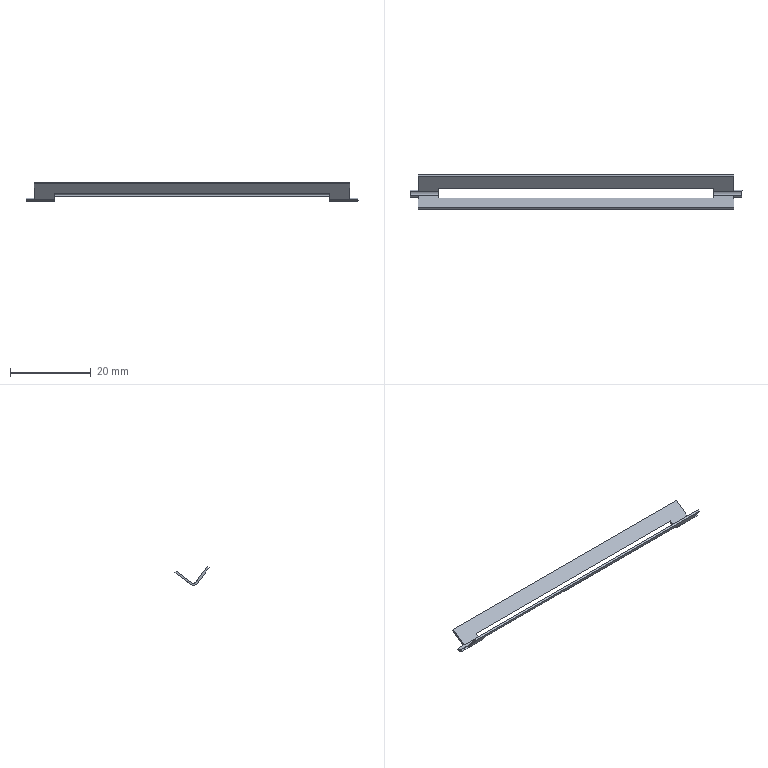Component | SolidWorks | ToolHolderAssembly-1_Blade-1 | 1 solid | 28 faces | box 82 x 8.4 x 4.59 mm | volume 284 mm3 | plane 24 | cylinder 4 | commonest cylinder face diameters 1.5 x2 2.5 x2
STEP:
#1=COLOUR_RGB('',0.7922,0.8196,0.9333);
#2=FILL_AREA_STYLE_COLOUR('',#1);
#3=FILL_AREA_STYLE('',(#2));
#4=SURFACE_STYLE_FILL_AREA(#3);
#5=SURFACE_SIDE_STYLE('',(#4));
#6=SURFACE_STYLE_USAGE(.BOTH.,#5);
#7=PRESENTATION_STYLE_ASSIGNMENT((#6));
#8=CARTESIAN_POINT('',(-4.579,0.3269,5.509));
#9=VERTEX_POINT('',#8);
#10=CARTESIAN_POINT('',(-7.257,0.3269,5.509));
#11=VERTEX_POINT('',#10);
#12=CARTESIAN_POINT('',(-7.257,0.3269,5.509));
#13=DIRECTION('',(-1.,0.,-0.));
#14=VECTOR('',#13,39.37);
#15=LINE('',#12,#14);
#16=EDGE_CURVE('',#9,#11,#15,.T.);
#17=ORIENTED_EDGE('',*,*,#16,.T.);
#18=CARTESIAN_POINT('',(-7.257,0.268,5.465));
#19=VERTEX_POINT('',#18);
#20=CARTESIAN_POINT('',(-7.257,0.2954,5.486));
#21=DIRECTION('',(0.,-0.799,-0.6013));
#22=VECTOR('',#21,39.37);
#23=LINE('',#20,#22);
#24=EDGE_CURVE('',#11,#19,#23,.T.);
#25=ORIENTED_EDGE('',*,*,#24,.T.);
#26=CARTESIAN_POINT('',(-7.453,0.268,5.465));
#27=VERTEX_POINT('',#26);
#28=CARTESIAN_POINT('',(-4.304,0.268,5.465));
#29=DIRECTION('',(-1.,0.,-0.));
#30=VECTOR('',#29,39.37);
#31=LINE('',#28,#30);
#32=EDGE_CURVE('',#19,#27,#31,.T.);
#33=ORIENTED_EDGE('',*,*,#32,.T.);
#34=CARTESIAN_POINT('',(-7.453,0.4174,5.577));
#35=VERTEX_POINT('',#34);
#36=CARTESIAN_POINT('',(-7.453,0.4174,5.577));
#37=DIRECTION('',(0.,-0.799,-0.6013));
#38=VECTOR('',#37,39.37);
#39=LINE('',#36,#38);
#40=EDGE_CURVE('',#35,#27,#39,.T.);
#41=ORIENTED_EDGE('',*,*,#40,.F.);
#42=CARTESIAN_POINT('',(-4.383,0.4174,5.577));
#43=VERTEX_POINT('',#42);
#44=CARTESIAN_POINT('',(-4.304,0.4174,5.577));
#45=DIRECTION('',(-1.,0.,-0.));
#46=VECTOR('',#45,39.37);
#47=LINE('',#44,#46);
#48=EDGE_CURVE('',#43,#35,#47,.T.);
#49=ORIENTED_EDGE('',*,*,#48,.F.);
#50=CARTESIAN_POINT('',(-4.383,0.268,5.465));
#51=VERTEX_POINT('',#50);
#52=CARTESIAN_POINT('',(-4.383,0.268,5.465));
#53=DIRECTION('',(-0.,0.799,0.6013));
#54=VECTOR('',#53,39.37);
#55=LINE('',#52,#54);
#56=EDGE_CURVE('',#51,#43,#55,.T.);
#57=ORIENTED_EDGE('',*,*,#56,.F.);
#58=CARTESIAN_POINT('',(-4.579,0.268,5.465));
#59=VERTEX_POINT('',#58);
#60=CARTESIAN_POINT('',(-4.304,0.268,5.465));
#61=DIRECTION('',(-1.,0.,-0.));
#62=VECTOR('',#61,39.37);
#63=LINE('',#60,#62);
#64=EDGE_CURVE('',#51,#59,#63,.T.);
#65=ORIENTED_EDGE('',*,*,#64,.T.);
#66=CARTESIAN_POINT('',(-4.579,0.1912,5.407));
#67=DIRECTION('',(-0.,0.799,0.6013));
#68=VECTOR('',#67,39.37);
#69=LINE('',#66,#68);
#70=EDGE_CURVE('',#59,#9,#69,.T.);
#71=ORIENTED_EDGE('',*,*,#70,.T.);
#72=EDGE_LOOP('',(#17,#25,#33,#41,#49,#57,#65,#71));
#73=FACE_OUTER_BOUND('',#72,.T.);
#74=CARTESIAN_POINT('',(-4.304,0.268,5.465));
#75=DIRECTION('',(-0.,-0.6013,0.799));
#76=DIRECTION('',(1.,-0.,0.));
#77=AXIS2_PLACEMENT_3D('',#74,#75,#76);
#78=PLANE('',#77);
#79=ADVANCED_FACE('',(#73),#78,.F.);
#80=CARTESIAN_POINT('',(-7.257,0.2878,5.505));
#81=VERTEX_POINT('',#80);
#82=CARTESIAN_POINT('',(-7.257,0.2562,5.481));
#83=VERTEX_POINT('',#82);
#84=CARTESIAN_POINT('',(-7.257,0.2315,5.462));
#85=DIRECTION('',(0.,-0.799,-0.6013));
#86=VECTOR('',#85,39.37);
#87=LINE('',#84,#86);
#88=EDGE_CURVE('',#81,#83,#87,.T.);
#89=ORIENTED_EDGE('',*,*,#88,.F.);
#90=CARTESIAN_POINT('',(-4.579,0.2878,5.505));
#91=VERTEX_POINT('',#90);
#92=CARTESIAN_POINT('',(-4.304,0.2878,5.505));
#93=DIRECTION('',(1.,-0.,0.));
#94=VECTOR('',#93,39.37);
#95=LINE('',#92,#94);
#96=EDGE_CURVE('',#81,#91,#95,.T.);
#97=ORIENTED_EDGE('',*,*,#96,.T.);
#98=CARTESIAN_POINT('',(-4.579,0.2562,5.481));
#99=VERTEX_POINT('',#98);
#100=CARTESIAN_POINT('',(-4.579,0.2315,5.462));
#101=DIRECTION('',(-0.,0.799,0.6013));
#102=VECTOR('',#101,39.37);
#103=LINE('',#100,#102);
#104=EDGE_CURVE('',#99,#91,#103,.T.);
#105=ORIENTED_EDGE('',*,*,#104,.F.);
#106=CARTESIAN_POINT('',(-4.383,0.2562,5.481));
#107=VERTEX_POINT('',#106);
#108=CARTESIAN_POINT('',(-4.304,0.2562,5.481));
#109=DIRECTION('',(-1.,0.,-0.));
#110=VECTOR('',#109,39.37);
#111=LINE('',#108,#110);
#112=EDGE_CURVE('',#107,#99,#111,.T.);
#113=ORIENTED_EDGE('',*,*,#112,.F.);
#114=CARTESIAN_POINT('',(-4.383,0.4056,5.593));
#115=VERTEX_POINT('',#114);
#116=CARTESIAN_POINT('',(-4.383,0.4056,5.593));
#117=DIRECTION('',(0.,-0.799,-0.6013));
#118=VECTOR('',#117,39.37);
#119=LINE('',#116,#118);
#120=EDGE_CURVE('',#115,#107,#119,.T.);
#121=ORIENTED_EDGE('',*,*,#120,.F.);
#122=CARTESIAN_POINT('',(-7.453,0.4056,5.593));
#123=VERTEX_POINT('',#122);
#124=CARTESIAN_POINT('',(-4.304,0.4056,5.593));
#125=DIRECTION('',(-1.,0.,-0.));
#126=VECTOR('',#125,39.37);
#127=LINE('',#124,#126);
#128=EDGE_CURVE('',#115,#123,#127,.T.);
#129=ORIENTED_EDGE('',*,*,#128,.T.);
#130=CARTESIAN_POINT('',(-7.453,0.2562,5.481));
#131=VERTEX_POINT('',#130);
#132=CARTESIAN_POINT('',(-7.453,0.2562,5.481));
#133=DIRECTION('',(-0.,0.799,0.6013));
#134=VECTOR('',#133,39.37);
#135=LINE('',#132,#134);
#136=EDGE_CURVE('',#131,#123,#135,.T.);
#137=ORIENTED_EDGE('',*,*,#136,.F.);
#138=CARTESIAN_POINT('',(-4.304,0.2562,5.481));
#139=DIRECTION('',(-1.,0.,-0.));
#140=VECTOR('',#139,39.37);
#141=LINE('',#138,#140);
#142=EDGE_CURVE('',#83,#131,#141,.T.);
#143=ORIENTED_EDGE('',*,*,#142,.F.);
#144=EDGE_LOOP('',(#89,#97,#105,#113,#121,#129,#137,#143));
#145=FACE_OUTER_BOUND('',#144,.T.);
#146=CARTESIAN_POINT('',(-4.304,0.2562,5.481));
#147=DIRECTION('',(-0.,-0.6013,0.799));
#148=DIRECTION('',(1.,-0.,0.));
#149=AXIS2_PLACEMENT_3D('',#146,#147,#148);
#150=PLANE('',#149);
#151=ADVANCED_FACE('',(#145),#150,.T.);
#152=CARTESIAN_POINT('',(-4.579,0.191,5.518));
#153=VERTEX_POINT('',#152);
#154=CARTESIAN_POINT('',(-4.579,0.2148,5.487));
#155=VERTEX_POINT('',#154);
#156=CARTESIAN_POINT('',(-4.579,0.2334,5.462));
#157=DIRECTION('',(0.,0.6013,-0.799));
#158=VECTOR('',#157,39.37);
#159=LINE('',#156,#158);
#160=EDGE_CURVE('',#153,#155,#159,.T.);
#161=ORIENTED_EDGE('',*,*,#160,.F.);
#162=CARTESIAN_POINT('',(-7.257,0.191,5.518));
#163=VERTEX_POINT('',#162);
#164=CARTESIAN_POINT('',(-4.304,0.191,5.518));
#165=DIRECTION('',(-1.,0.,-0.));
#166=VECTOR('',#165,39.37);
#167=LINE('',#164,#166);
#168=EDGE_CURVE('',#153,#163,#167,.T.);
#169=ORIENTED_EDGE('',*,*,#168,.T.);
#170=CARTESIAN_POINT('',(-7.257,0.2148,5.487));
#171=VERTEX_POINT('',#170);
#172=CARTESIAN_POINT('',(-7.257,0.2334,5.462));
#173=DIRECTION('',(-0.,-0.6013,0.799));
#174=VECTOR('',#173,39.37);
#175=LINE('',#172,#174);
#176=EDGE_CURVE('',#171,#163,#175,.T.);
#177=ORIENTED_EDGE('',*,*,#176,.F.);
#178=CARTESIAN_POINT('',(-7.453,0.2148,5.487));
#179=VERTEX_POINT('',#178);
#180=CARTESIAN_POINT('',(-4.304,0.2148,5.487));
#181=DIRECTION('',(-1.,0.,-0.));
#182=VECTOR('',#181,39.37);
#183=LINE('',#180,#182);
#184=EDGE_CURVE('',#171,#179,#183,.T.);
#185=ORIENTED_EDGE('',*,*,#184,.T.);
#186=CARTESIAN_POINT('',(-7.453,0.1024,5.636));
#187=VERTEX_POINT('',#186);
#188=CARTESIAN_POINT('',(-7.453,0.1024,5.636));
#189=DIRECTION('',(0.,0.6013,-0.799));
#190=VECTOR('',#189,39.37);
#191=LINE('',#188,#190);
#192=EDGE_CURVE('',#187,#179,#191,.T.);
#193=ORIENTED_EDGE('',*,*,#192,.F.);
#194=CARTESIAN_POINT('',(-4.383,0.1024,5.636));
#195=VERTEX_POINT('',#194);
#196=CARTESIAN_POINT('',(-4.304,0.1024,5.636));
#197=DIRECTION('',(-1.,0.,-0.));
#198=VECTOR('',#197,39.37);
#199=LINE('',#196,#198);
#200=EDGE_CURVE('',#195,#187,#199,.T.);
#201=ORIENTED_EDGE('',*,*,#200,.F.);
#202=CARTESIAN_POINT('',(-4.383,0.2148,5.487));
#203=VERTEX_POINT('',#202);
#204=CARTESIAN_POINT('',(-4.383,0.2148,5.487));
#205=DIRECTION('',(-0.,-0.6013,0.799));
#206=VECTOR('',#205,39.37);
#207=LINE('',#204,#206);
#208=EDGE_CURVE('',#203,#195,#207,.T.);
#209=ORIENTED_EDGE('',*,*,#208,.F.);
#210=CARTESIAN_POINT('',(-4.304,0.2148,5.487));
#211=DIRECTION('',(-1.,0.,-0.));
#212=VECTOR('',#211,39.37);
#213=LINE('',#210,#212);
#214=EDGE_CURVE('',#203,#155,#213,.T.);
#215=ORIENTED_EDGE('',*,*,#214,.T.);
#216=EDGE_LOOP('',(#161,#169,#177,#185,#193,#201,#209,#215));
#217=FACE_OUTER_BOUND('',#216,.T.);
#218=CARTESIAN_POINT('',(-4.304,0.1024,5.636));
#219=DIRECTION('',(-0.,0.799,0.6013));
#220=DIRECTION('',(-1.,0.,-0.));
#221=AXIS2_PLACEMENT_3D('',#218,#219,#220);
#222=PLANE('',#221);
#223=ADVANCED_FACE('',(#217),#222,.T.);
#224=CARTESIAN_POINT('',(-7.257,0.1548,5.534));
#225=VERTEX_POINT('',#224);
#226=CARTESIAN_POINT('',(-4.579,0.1548,5.534));
#227=VERTEX_POINT('',#226);
#228=CARTESIAN_POINT('',(-4.579,0.1548,5.534));
#229=DIRECTION('',(1.,-0.,0.));
#230=VECTOR('',#229,39.37);
#231=LINE('',#228,#230);
#232=EDGE_CURVE('',#225,#227,#231,.T.);
#233=ORIENTED_EDGE('',*,*,#232,.T.);
#234=CARTESIAN_POINT('',(-4.579,0.1991,5.475));
#235=VERTEX_POINT('',#234);
#236=CARTESIAN_POINT('',(-4.579,0.1785,5.502));
#237=DIRECTION('',(0.,0.6013,-0.799));
#238=VECTOR('',#237,39.37);
#239=LINE('',#236,#238);
#240=EDGE_CURVE('',#227,#235,#239,.T.);
#241=ORIENTED_EDGE('',*,*,#240,.T.);
#242=CARTESIAN_POINT('',(-4.383,0.1991,5.475));
#243=VERTEX_POINT('',#242);
#244=CARTESIAN_POINT('',(-4.304,0.1991,5.475));
#245=DIRECTION('',(-1.,0.,-0.));
#246=VECTOR('',#245,39.37);
#247=LINE('',#244,#246);
#248=EDGE_CURVE('',#243,#235,#247,.T.);
#249=ORIENTED_EDGE('',*,*,#248,.F.);
#250=CARTESIAN_POINT('',(-4.383,0.08665,5.624));
#251=VERTEX_POINT('',#250);
#252=CARTESIAN_POINT('',(-4.383,0.08665,5.624));
#253=DIRECTION('',(0.,0.6013,-0.799));
#254=VECTOR('',#253,39.37);
#255=LINE('',#252,#254);
#256=EDGE_CURVE('',#251,#243,#255,.T.);
#257=ORIENTED_EDGE('',*,*,#256,.F.);
#258=CARTESIAN_POINT('',(-7.453,0.08665,5.624));
#259=VERTEX_POINT('',#258);
#260=CARTESIAN_POINT('',(-4.304,0.08665,5.624));
#261=DIRECTION('',(-1.,0.,-0.));
#262=VECTOR('',#261,39.37);
#263=LINE('',#260,#262);
#264=EDGE_CURVE('',#251,#259,#263,.T.);
#265=ORIENTED_EDGE('',*,*,#264,.T.);
#266=CARTESIAN_POINT('',(-7.453,0.1991,5.475));
#267=VERTEX_POINT('',#266);
#268=CARTESIAN_POINT('',(-7.453,0.1991,5.475));
#269=DIRECTION('',(-0.,-0.6013,0.799));
#270=VECTOR('',#269,39.37);
#271=LINE('',#268,#270);
#272=EDGE_CURVE('',#267,#259,#271,.T.);
#273=ORIENTED_EDGE('',*,*,#272,.F.);
#274=CARTESIAN_POINT('',(-7.257,0.1991,5.475));
#275=VERTEX_POINT('',#274);
#276=CARTESIAN_POINT('',(-4.304,0.1991,5.475));
#277=DIRECTION('',(-1.,0.,-0.));
#278=VECTOR('',#277,39.37);
#279=LINE('',#276,#278);
#280=EDGE_CURVE('',#275,#267,#279,.T.);
#281=ORIENTED_EDGE('',*,*,#280,.F.);
#282=CARTESIAN_POINT('',(-7.257,0.2569,5.398));
#283=DIRECTION('',(-0.,-0.6013,0.799));
#284=VECTOR('',#283,39.37);
#285=LINE('',#282,#284);
#286=EDGE_CURVE('',#275,#225,#285,.T.);
#287=ORIENTED_EDGE('',*,*,#286,.T.);
#288=EDGE_LOOP('',(#233,#241,#249,#257,#265,#273,#281,#287));
#289=FACE_OUTER_BOUND('',#288,.T.);
#290=CARTESIAN_POINT('',(-4.304,0.08665,5.624));
#291=DIRECTION('',(-0.,0.799,0.6013));
#292=DIRECTION('',(-1.,0.,-0.));
#293=AXIS2_PLACEMENT_3D('',#290,#291,#292);
#294=PLANE('',#293);
#295=ADVANCED_FACE('',(#289),#294,.F.);
#296=ORIENTED_EDGE('',*,*,#184,.F.);
#297=CARTESIAN_POINT('',(-7.257,0.2384,5.504));
#298=DIRECTION('',(1.,-0.,0.));
#299=DIRECTION('',(0.,-0.799,-0.6013));
#300=AXIS2_PLACEMENT_3D('',#297,#298,#299);
#301=CIRCLE('',#300,0.02953);
#302=EDGE_CURVE('',#171,#83,#301,.T.);
#303=ORIENTED_EDGE('',*,*,#302,.T.);
#304=ORIENTED_EDGE('',*,*,#142,.T.);
#305=CARTESIAN_POINT('',(-7.532,0.2562,5.481));
#306=VERTEX_POINT('',#305);
#307=CARTESIAN_POINT('',(-7.453,0.2562,5.481));
#308=DIRECTION('',(-1.,0.,-0.));
#309=VECTOR('',#308,39.37);
#310=LINE('',#307,#309);
#311=EDGE_CURVE('',#131,#306,#310,.T.);
#312=ORIENTED_EDGE('',*,*,#311,.T.);
#313=CARTESIAN_POINT('',(-7.532,0.2148,5.487));
#314=VERTEX_POINT('',#313);
#315=CARTESIAN_POINT('',(-7.532,0.2384,5.504));
#316=DIRECTION('',(1.,-0.,0.));
#317=DIRECTION('',(0.,0.799,0.6013));
#318=AXIS2_PLACEMENT_3D('',#315,#316,#317);
#319=CIRCLE('',#318,0.02953);
#320=EDGE_CURVE('',#314,#306,#319,.T.);
#321=ORIENTED_EDGE('',*,*,#320,.F.);
#322=CARTESIAN_POINT('',(-7.453,0.2148,5.487));
#323=DIRECTION('',(-1.,0.,-0.));
#324=VECTOR('',#323,39.37);
#325=LINE('',#322,#324);
#326=EDGE_CURVE('',#179,#314,#325,.T.);
#327=ORIENTED_EDGE('',*,*,#326,.F.);
#328=EDGE_LOOP('',(#296,#303,#304,#312,#321,#327));
#329=FACE_OUTER_BOUND('',#328,.T.);
#330=CARTESIAN_POINT('',(-4.304,0.2384,5.504));
#331=DIRECTION('',(-1.,0.,-0.));
#332=DIRECTION('',(0.,-0.799,-0.6013));
#333=AXIS2_PLACEMENT_3D('',#330,#331,#332);
#334=CYLINDRICAL_SURFACE('',#333,0.02953);
#335=ADVANCED_FACE('',(#329),#334,.F.);
#336=ORIENTED_EDGE('',*,*,#112,.T.);
#337=CARTESIAN_POINT('',(-4.579,0.2384,5.504));
#338=DIRECTION('',(-1.,0.,-0.));
#339=DIRECTION('',(0.,0.799,0.6013));
#340=AXIS2_PLACEMENT_3D('',#337,#338,#339);
#341=CIRCLE('',#340,0.02953);
#342=EDGE_CURVE('',#99,#155,#341,.T.);
#343=ORIENTED_EDGE('',*,*,#342,.T.);
#344=ORIENTED_EDGE('',*,*,#214,.F.);
#345=CARTESIAN_POINT('',(-4.304,0.2148,5.487));
#346=VERTEX_POINT('',#345);
#347=CARTESIAN_POINT('',(-4.304,0.2148,5.487));
#348=DIRECTION('',(-1.,0.,-0.));
#349=VECTOR('',#348,39.37);
#350=LINE('',#347,#349);
#351=EDGE_CURVE('',#346,#203,#350,.T.);
#352=ORIENTED_EDGE('',*,*,#351,.F.);
#353=CARTESIAN_POINT('',(-4.304,0.2562,5.481));
#354=VERTEX_POINT('',#353);
#355=CARTESIAN_POINT('',(-4.304,0.2384,5.504));
#356=DIRECTION('',(1.,-0.,0.));
#357=DIRECTION('',(0.,0.799,0.6013));
#358=AXIS2_PLACEMENT_3D('',#355,#356,#357);
#359=CIRCLE('',#358,0.02953);
#360=EDGE_CURVE('',#346,#354,#359,.T.);
#361=ORIENTED_EDGE('',*,*,#360,.T.);
#362=CARTESIAN_POINT('',(-4.304,0.2562,5.481));
#363=DIRECTION('',(-1.,0.,-0.));
#364=VECTOR('',#363,39.37);
#365=LINE('',#362,#364);
#366=EDGE_CURVE('',#354,#107,#365,.T.);
#367=ORIENTED_EDGE('',*,*,#366,.T.);
#368=EDGE_LOOP('',(#336,#343,#344,#352,#361,#367));
#369=FACE_OUTER_BOUND('',#368,.T.);
#370=CARTESIAN_POINT('',(-4.304,0.2384,5.504));
#371=DIRECTION('',(-1.,0.,-0.));
#372=DIRECTION('',(0.,-0.799,-0.6013));
#373=AXIS2_PLACEMENT_3D('',#370,#371,#372);
#374=CYLINDRICAL_SURFACE('',#373,0.02953);
#375=ADVANCED_FACE('',(#369),#374,.F.);
#376=CARTESIAN_POINT('',(-7.257,0.2384,5.504));
#377=DIRECTION('',(1.,-0.,0.));
#378=DIRECTION('',(0.,-0.799,-0.6013));
#379=AXIS2_PLACEMENT_3D('',#376,#377,#378);
#380=CIRCLE('',#379,0.04921);
#381=EDGE_CURVE('',#275,#19,#380,.T.);
#382=ORIENTED_EDGE('',*,*,#381,.F.);
#383=ORIENTED_EDGE('',*,*,#280,.T.);
#384=CARTESIAN_POINT('',(-7.532,0.1991,5.475));
#385=VERTEX_POINT('',#384);
#386=CARTESIAN_POINT('',(-7.453,0.1991,5.475));
#387=DIRECTION('',(-1.,0.,-0.));
#388=VECTOR('',#387,39.37);
#389=LINE('',#386,#388);
#390=EDGE_CURVE('',#267,#385,#389,.T.);
#391=ORIENTED_EDGE('',*,*,#390,.T.);
#392=CARTESIAN_POINT('',(-7.532,0.268,5.465));
#393=VERTEX_POINT('',#392);
#394=CARTESIAN_POINT('',(-7.532,0.2384,5.504));
#395=DIRECTION('',(1.,-0.,0.));
#396=DIRECTION('',(0.,-0.799,-0.6013));
#397=AXIS2_PLACEMENT_3D('',#394,#395,#396);
#398=CIRCLE('',#397,0.04921);
#399=EDGE_CURVE('',#385,#393,#398,.T.);
#400=ORIENTED_EDGE('',*,*,#399,.T.);
#401=CARTESIAN_POINT('',(-7.453,0.268,5.465));
#402=DIRECTION('',(-1.,0.,-0.));
#403=VECTOR('',#402,39.37);
#404=LINE('',#401,#403);
#405=EDGE_CURVE('',#27,#393,#404,.T.);
#406=ORIENTED_EDGE('',*,*,#405,.F.);
#407=ORIENTED_EDGE('',*,*,#32,.F.);
#408=EDGE_LOOP('',(#382,#383,#391,#400,#406,#407));
#409=FACE_OUTER_BOUND('',#408,.T.);
#410=CARTESIAN_POINT('',(-4.304,0.2384,5.504));
#411=DIRECTION('',(-1.,0.,-0.));
#412=DIRECTION('',(0.,-0.799,-0.6013));
#413=AXIS2_PLACEMENT_3D('',#410,#411,#412);
#414=CYLINDRICAL_SURFACE('',#413,0.04921);
#415=ADVANCED_FACE('',(#409),#414,.T.);
#416=CARTESIAN_POINT('',(-4.579,0.2384,5.504));
#417=DIRECTION('',(-1.,0.,-0.));
#418=DIRECTION('',(0.,-0.799,-0.6013));
#419=AXIS2_PLACEMENT_3D('',#416,#417,#418);
#420=CIRCLE('',#419,0.04921);
#421=EDGE_CURVE('',#59,#235,#420,.T.);
#422=ORIENTED_EDGE('',*,*,#421,.F.);
#423=ORIENTED_EDGE('',*,*,#64,.F.);
#424=CARTESIAN_POINT('',(-4.304,0.268,5.465));
#425=VERTEX_POINT('',#424);
#426=CARTESIAN_POINT('',(-4.304,0.268,5.465));
#427=DIRECTION('',(-1.,0.,-0.));
#428=VECTOR('',#427,39.37);
#429=LINE('',#426,#428);
#430=EDGE_CURVE('',#425,#51,#429,.T.);
#431=ORIENTED_EDGE('',*,*,#430,.F.);
#432=CARTESIAN_POINT('',(-4.304,0.1991,5.475));
#433=VERTEX_POINT('',#432);
#434=CARTESIAN_POINT('',(-4.304,0.2384,5.504));
#435=DIRECTION('',(1.,-0.,0.));
#436=DIRECTION('',(0.,-0.799,-0.6013));
#437=AXIS2_PLACEMENT_3D('',#434,#435,#436);
#438=CIRCLE('',#437,0.04921);
#439=EDGE_CURVE('',#433,#425,#438,.T.);
#440=ORIENTED_EDGE('',*,*,#439,.F.);
#441=CARTESIAN_POINT('',(-4.304,0.1991,5.475));
#442=DIRECTION('',(-1.,0.,-0.));
#443=VECTOR('',#442,39.37);
#444=LINE('',#441,#443);
#445=EDGE_CURVE('',#433,#243,#444,.T.);
#446=ORIENTED_EDGE('',*,*,#445,.T.);
#447=ORIENTED_EDGE('',*,*,#248,.T.);
#448=EDGE_LOOP('',(#422,#423,#431,#440,#446,#447));
#449=FACE_OUTER_BOUND('',#448,.T.);
#450=CARTESIAN_POINT('',(-4.304,0.2384,5.504));
#451=DIRECTION('',(-1.,0.,-0.));
#452=DIRECTION('',(0.,-0.799,-0.6013));
#453=AXIS2_PLACEMENT_3D('',#450,#451,#452);
#454=CYLINDRICAL_SURFACE('',#453,0.04921);
#455=ADVANCED_FACE('',(#449),#454,.T.);
#456=ORIENTED_EDGE('',*,*,#48,.T.);
#457=CARTESIAN_POINT('',(-7.453,0.4056,5.593));
#458=DIRECTION('',(0.,0.6013,-0.799));
#459=VECTOR('',#458,39.37);
#460=LINE('',#457,#459);
#461=EDGE_CURVE('',#123,#35,#460,.T.);
#462=ORIENTED_EDGE('',*,*,#461,.F.);
#463=ORIENTED_EDGE('',*,*,#128,.F.);
#464=CARTESIAN_POINT('',(-4.383,0.4174,5.577));
#465=DIRECTION('',(-0.,-0.6013,0.799));
#466=VECTOR('',#465,39.37);
#467=LINE('',#464,#466);
#468=EDGE_CURVE('',#43,#115,#467,.T.);
#469=ORIENTED_EDGE('',*,*,#468,.F.);
#470=EDGE_LOOP('',(#456,#462,#463,#469));
#471=FACE_OUTER_BOUND('',#470,.T.);
#472=CARTESIAN_POINT('',(-4.304,0.4056,5.593));
#473=DIRECTION('',(-0.,0.799,0.6013));
#474=DIRECTION('',(-1.,0.,-0.));
#475=AXIS2_PLACEMENT_3D('',#472,#473,#474);
#476=PLANE('',#475);
#477=ADVANCED_FACE('',(#471),#476,.T.);
#478=ORIENTED_EDGE('',*,*,#200,.T.);
#479=CARTESIAN_POINT('',(-7.453,0.08665,5.624));
#480=DIRECTION('',(-0.,0.799,0.6013));
#481=VECTOR('',#480,39.37);
#482=LINE('',#479,#481);
#483=EDGE_CURVE('',#259,#187,#482,.T.);
#484=ORIENTED_EDGE('',*,*,#483,.F.);
#485=ORIENTED_EDGE('',*,*,#264,.F.);
#486=CARTESIAN_POINT('',(-4.383,0.1024,5.636));
#487=DIRECTION('',(0.,-0.799,-0.6013));
#488=VECTOR('',#487,39.37);
#489=LINE('',#486,#488);
#490=EDGE_CURVE('',#195,#251,#489,.T.);
#491=ORIENTED_EDGE('',*,*,#490,.F.);
#492=EDGE_LOOP('',(#478,#484,#485,#491));
#493=FACE_OUTER_BOUND('',#492,.T.);
#494=CARTESIAN_POINT('',(-4.304,0.08665,5.624));
#495=DIRECTION('',(-0.,-0.6013,0.799));
#496=DIRECTION('',(1.,-0.,0.));
#497=AXIS2_PLACEMENT_3D('',#494,#495,#496);
#498=PLANE('',#497);
#499=ADVANCED_FACE('',(#493),#498,.T.);
#500=CARTESIAN_POINT('',(-4.304,0.1991,5.475));
#501=DIRECTION('',(-0.,0.799,0.6013));
#502=VECTOR('',#501,39.37);
#503=LINE('',#500,#502);
#504=EDGE_CURVE('',#433,#346,#503,.T.);
#505=ORIENTED_EDGE('',*,*,#504,.F.);
#506=ORIENTED_EDGE('',*,*,#439,.T.);
#507=CARTESIAN_POINT('',(-4.304,0.2562,5.481));
#508=DIRECTION('',(0.,0.6013,-0.799));
#509=VECTOR('',#508,39.37);
#510=LINE('',#507,#509);
#511=EDGE_CURVE('',#354,#425,#510,.T.);
#512=ORIENTED_EDGE('',*,*,#511,.F.);
#513=ORIENTED_EDGE('',*,*,#360,.F.);
#514=EDGE_LOOP('',(#505,#506,#512,#513));
#515=FACE_OUTER_BOUND('',#514,.T.);
#516=CARTESIAN_POINT('',(-4.304,0.1991,5.475));
#517=DIRECTION('',(1.,-0.,0.));
#518=DIRECTION('',(-0.,0.799,0.6013));
#519=AXIS2_PLACEMENT_3D('',#516,#517,#518);
#520=PLANE('',#519);
#521=ADVANCED_FACE('',(#515),#520,.T.);
#522=CARTESIAN_POINT('',(-7.532,0.268,5.465));
#523=DIRECTION('',(-0.,-0.6013,0.799));
#524=VECTOR('',#523,39.37);
#525=LINE('',#522,#524);
#526=EDGE_CURVE('',#393,#306,#525,.T.);
#527=ORIENTED_EDGE('',*,*,#526,.F.);
#528=ORIENTED_EDGE('',*,*,#399,.F.);
#529=CARTESIAN_POINT('',(-7.532,0.2148,5.487));
#530=DIRECTION('',(0.,-0.799,-0.6013));
#531=VECTOR('',#530,39.37);
#532=LINE('',#529,#531);
#533=EDGE_CURVE('',#314,#385,#532,.T.);
#534=ORIENTED_EDGE('',*,*,#533,.F.);
#535=ORIENTED_EDGE('',*,*,#320,.T.);
#536=EDGE_LOOP('',(#527,#528,#534,#535));
#537=FACE_OUTER_BOUND('',#536,.T.);
#538=CARTESIAN_POINT('',(-7.532,0.268,5.465));
#539=DIRECTION('',(-1.,0.,-0.));
#540=DIRECTION('',(0.,-0.799,-0.6013));
#541=AXIS2_PLACEMENT_3D('',#538,#539,#540);
#542=PLANE('',#541);
#543=ADVANCED_FACE('',(#537),#542,.T.);
#544=ORIENTED_EDGE('',*,*,#511,.T.);
#545=ORIENTED_EDGE('',*,*,#430,.T.);
#546=CARTESIAN_POINT('',(-4.383,0.2562,5.481));
#547=DIRECTION('',(0.,0.6013,-0.799));
#548=VECTOR('',#547,39.37);
#549=LINE('',#546,#548);
#550=EDGE_CURVE('',#107,#51,#549,.T.);
#551=ORIENTED_EDGE('',*,*,#550,.F.);
#552=ORIENTED_EDGE('',*,*,#366,.F.);
#553=EDGE_LOOP('',(#544,#545,#551,#552));
#554=FACE_OUTER_BOUND('',#553,.T.);
#555=CARTESIAN_POINT('',(-4.383,0.2562,5.481));
#556=DIRECTION('',(0.,-0.799,-0.6013));
#557=DIRECTION('',(1.,-0.,0.));
#558=AXIS2_PLACEMENT_3D('',#555,#556,#557);
#559=PLANE('',#558);
#560=ADVANCED_FACE('',(#554),#559,.F.);
#561=ORIENTED_EDGE('',*,*,#550,.T.);
#562=ORIENTED_EDGE('',*,*,#56,.T.);
#563=ORIENTED_EDGE('',*,*,#468,.T.);
#564=ORIENTED_EDGE('',*,*,#120,.T.);
#565=EDGE_LOOP('',(#561,#562,#563,#564));
#566=FACE_OUTER_BOUND('',#565,.T.);
#567=CARTESIAN_POINT('',(-4.383,0.2287,5.435));
#568=DIRECTION('',(1.,-0.,0.));
#569=DIRECTION('',(-0.,0.799,0.6013));
#570=AXIS2_PLACEMENT_3D('',#567,#568,#569);
#571=PLANE('',#570);
#572=ADVANCED_FACE('',(#566),#571,.T.);
#573=ORIENTED_EDGE('',*,*,#504,.T.);
#574=ORIENTED_EDGE('',*,*,#351,.T.);
#575=CARTESIAN_POINT('',(-4.383,0.1991,5.475));
#576=DIRECTION('',(-0.,0.799,0.6013));
#577=VECTOR('',#576,39.37);
#578=LINE('',#575,#577);
#579=EDGE_CURVE('',#243,#203,#578,.T.);
#580=ORIENTED_EDGE('',*,*,#579,.F.);
#581=ORIENTED_EDGE('',*,*,#445,.F.);
#582=EDGE_LOOP('',(#573,#574,#580,#581));
#583=FACE_OUTER_BOUND('',#582,.T.);
#584=CARTESIAN_POINT('',(-4.383,0.1991,5.475));
#585=DIRECTION('',(0.,0.6013,-0.799));
#586=DIRECTION('',(-0.,0.799,0.6013));
#587=AXIS2_PLACEMENT_3D('',#584,#585,#586);
#588=PLANE('',#587);
#589=ADVANCED_FACE('',(#583),#588,.F.);
#590=ORIENTED_EDGE('',*,*,#490,.T.);
#591=ORIENTED_EDGE('',*,*,#256,.T.);
#592=ORIENTED_EDGE('',*,*,#579,.T.);
#593=ORIENTED_EDGE('',*,*,#208,.T.);
#594=EDGE_LOOP('',(#590,#591,#592,#593));
#595=FACE_OUTER_BOUND('',#594,.T.);
#596=CARTESIAN_POINT('',(-4.383,0.2287,5.435));
#597=DIRECTION('',(1.,-0.,0.));
#598=DIRECTION('',(-0.,0.799,0.6013));
#599=AXIS2_PLACEMENT_3D('',#596,#597,#598);
#600=PLANE('',#599);
#601=ADVANCED_FACE('',(#595),#600,.T.);
#602=ORIENTED_EDGE('',*,*,#533,.T.);
#603=ORIENTED_EDGE('',*,*,#390,.F.);
#604=CARTESIAN_POINT('',(-7.453,0.2148,5.487));
#605=DIRECTION('',(0.,-0.799,-0.6013));
#606=VECTOR('',#605,39.37);
#607=LINE('',#604,#606);
#608=EDGE_CURVE('',#179,#267,#607,.T.);
#609=ORIENTED_EDGE('',*,*,#608,.F.);
#610=ORIENTED_EDGE('',*,*,#326,.T.);
#611=EDGE_LOOP('',(#602,#603,#609,#610));
#612=FACE_OUTER_BOUND('',#611,.T.);
#613=CARTESIAN_POINT('',(-7.453,0.2148,5.487));
#614=DIRECTION('',(0.,0.6013,-0.799));
#615=DIRECTION('',(-0.,0.799,0.6013));
#616=AXIS2_PLACEMENT_3D('',#613,#614,#615);
#617=PLANE('',#616);
#618=ADVANCED_FACE('',(#612),#617,.F.);
#619=ORIENTED_EDGE('',*,*,#483,.T.);
#620=ORIENTED_EDGE('',*,*,#192,.T.);
#621=ORIENTED_EDGE('',*,*,#608,.T.);
#622=ORIENTED_EDGE('',*,*,#272,.T.);
#623=EDGE_LOOP('',(#619,#620,#621,#622));
#624=FACE_OUTER_BOUND('',#623,.T.);
#625=CARTESIAN_POINT('',(-7.453,0.2287,5.435));
#626=DIRECTION('',(-1.,0.,-0.));
#627=DIRECTION('',(0.,-0.799,-0.6013));
#628=AXIS2_PLACEMENT_3D('',#625,#626,#627);
#629=PLANE('',#628);
#630=ADVANCED_FACE('',(#624),#629,.T.);
#631=ORIENTED_EDGE('',*,*,#526,.T.);
#632=ORIENTED_EDGE('',*,*,#311,.F.);
#633=CARTESIAN_POINT('',(-7.453,0.268,5.465));
#634=DIRECTION('',(-0.,-0.6013,0.799));
#635=VECTOR('',#634,39.37);
#636=LINE('',#633,#635);
#637=EDGE_CURVE('',#27,#131,#636,.T.);
#638=ORIENTED_EDGE('',*,*,#637,.F.);
#639=ORIENTED_EDGE('',*,*,#405,.T.);
#640=EDGE_LOOP('',(#631,#632,#638,#639));
#641=FACE_OUTER_BOUND('',#640,.T.);
#642=CARTESIAN_POINT('',(-7.453,0.268,5.465));
#643=DIRECTION('',(0.,-0.799,-0.6013));
#644=DIRECTION('',(1.,-0.,0.));
#645=AXIS2_PLACEMENT_3D('',#642,#643,#644);
#646=PLANE('',#645);
#647=ADVANCED_FACE('',(#641),#646,.F.);
#648=ORIENTED_EDGE('',*,*,#461,.T.);
#649=ORIENTED_EDGE('',*,*,#40,.T.);
#650=ORIENTED_EDGE('',*,*,#637,.T.);
#651=ORIENTED_EDGE('',*,*,#136,.T.);
#652=EDGE_LOOP('',(#648,#649,#650,#651));
#653=FACE_OUTER_BOUND('',#652,.T.);
#654=CARTESIAN_POINT('',(-7.453,0.2287,5.435));
#655=DIRECTION('',(-1.,0.,-0.));
#656=DIRECTION('',(0.,-0.799,-0.6013));
#657=AXIS2_PLACEMENT_3D('',#654,#655,#656);
#658=PLANE('',#657);
#659=ADVANCED_FACE('',(#653),#658,.T.);
#660=CARTESIAN_POINT('',(-7.257,0.2148,5.487));
#661=DIRECTION('',(0.,-0.799,-0.6013));
#662=VECTOR('',#661,39.37);
#663=LINE('',#660,#662);
#664=EDGE_CURVE('',#171,#275,#663,.T.);
#665=ORIENTED_EDGE('',*,*,#664,.T.);
#666=ORIENTED_EDGE('',*,*,#381,.T.);
#667=CARTESIAN_POINT('',(-7.257,0.268,5.465));
#668=DIRECTION('',(-0.,-0.6013,0.799));
#669=VECTOR('',#668,39.37);
#670=LINE('',#667,#669);
#671=EDGE_CURVE('',#19,#83,#670,.T.);
#672=ORIENTED_EDGE('',*,*,#671,.T.);
#673=ORIENTED_EDGE('',*,*,#302,.F.);
#674=EDGE_LOOP('',(#665,#666,#672,#673));
#675=FACE_OUTER_BOUND('',#674,.T.);
#676=CARTESIAN_POINT('',(-7.257,0.2384,5.504));
#677=DIRECTION('',(-1.,0.,-0.));
#678=DIRECTION('',(0.,-0.799,-0.6013));
#679=AXIS2_PLACEMENT_3D('',#676,#677,#678);
#680=PLANE('',#679);
#681=ADVANCED_FACE('',(#675),#680,.F.);
#682=CARTESIAN_POINT('',(-4.579,0.2562,5.481));
#683=DIRECTION('',(0.,0.6013,-0.799));
#684=VECTOR('',#683,39.37);
#685=LINE('',#682,#684);
#686=EDGE_CURVE('',#99,#59,#685,.T.);
#687=ORIENTED_EDGE('',*,*,#686,.T.);
#688=ORIENTED_EDGE('',*,*,#421,.T.);
#689=CARTESIAN_POINT('',(-4.579,0.1991,5.475));
#690=DIRECTION('',(-0.,0.799,0.6013));
#691=VECTOR('',#690,39.37);
#692=LINE('',#689,#691);
#693=EDGE_CURVE('',#235,#155,#692,.T.);
#694=ORIENTED_EDGE('',*,*,#693,.T.);
#695=ORIENTED_EDGE('',*,*,#342,.F.);
#696=EDGE_LOOP('',(#687,#688,#694,#695));
#697=FACE_OUTER_BOUND('',#696,.T.);
#698=CARTESIAN_POINT('',(-4.579,0.2384,5.504));
#699=DIRECTION('',(1.,-0.,0.));
#700=DIRECTION('',(-0.,0.799,0.6013));
#701=AXIS2_PLACEMENT_3D('',#698,#699,#700);
#702=PLANE('',#701);
#703=ADVANCED_FACE('',(#697),#702,.F.);
#704=ORIENTED_EDGE('',*,*,#664,.F.);
#705=ORIENTED_EDGE('',*,*,#176,.T.);
#706=CARTESIAN_POINT('',(-7.257,0.1548,5.534));
#707=DIRECTION('',(-0.,-0.9203,0.3913));
#708=VECTOR('',#707,39.37);
#709=LINE('',#706,#708);
#710=EDGE_CURVE('',#163,#225,#709,.T.);
#711=ORIENTED_EDGE('',*,*,#710,.T.);
#712=ORIENTED_EDGE('',*,*,#286,.F.);
#713=EDGE_LOOP('',(#704,#705,#711,#712));
#714=FACE_OUTER_BOUND('',#713,.T.);
#715=CARTESIAN_POINT('',(-7.257,0.2569,5.398));
#716=DIRECTION('',(-1.,0.,-0.));
#717=DIRECTION('',(-0.,-0.6013,0.799));
#718=AXIS2_PLACEMENT_3D('',#715,#716,#717);
#719=PLANE('',#718);
#720=ADVANCED_FACE('',(#714),#719,.F.);
#721=ORIENTED_EDGE('',*,*,#693,.F.);
#722=ORIENTED_EDGE('',*,*,#240,.F.);
#723=CARTESIAN_POINT('',(-4.579,0.1548,5.534));
#724=DIRECTION('',(0.,0.9203,-0.3913));
#725=VECTOR('',#724,39.37);
#726=LINE('',#723,#725);
#727=EDGE_CURVE('',#227,#153,#726,.T.);
#728=ORIENTED_EDGE('',*,*,#727,.T.);
#729=ORIENTED_EDGE('',*,*,#160,.T.);
#730=EDGE_LOOP('',(#721,#722,#728,#729));
#731=FACE_OUTER_BOUND('',#730,.T.);
#732=CARTESIAN_POINT('',(-4.579,0.1785,5.502));
#733=DIRECTION('',(1.,-0.,0.));
#734=DIRECTION('',(0.,0.6013,-0.799));
#735=AXIS2_PLACEMENT_3D('',#732,#733,#734);
#736=PLANE('',#735);
#737=ADVANCED_FACE('',(#731),#736,.F.);
#738=ORIENTED_EDGE('',*,*,#686,.F.);
#739=ORIENTED_EDGE('',*,*,#104,.T.);
#740=CARTESIAN_POINT('',(-4.579,0.3269,5.509));
#741=DIRECTION('',(0.,0.9926,0.1213));
#742=VECTOR('',#741,39.37);
#743=LINE('',#740,#742);
#744=EDGE_CURVE('',#91,#9,#743,.T.);
#745=ORIENTED_EDGE('',*,*,#744,.T.);
#746=ORIENTED_EDGE('',*,*,#70,.F.);
#747=EDGE_LOOP('',(#738,#739,#745,#746));
#748=FACE_OUTER_BOUND('',#747,.T.);
#749=CARTESIAN_POINT('',(-4.579,0.1912,5.407));
#750=DIRECTION('',(1.,-0.,0.));
#751=DIRECTION('',(-0.,0.799,0.6013));
#752=AXIS2_PLACEMENT_3D('',#749,#750,#751);
#753=PLANE('',#752);
#754=ADVANCED_FACE('',(#748),#753,.F.);
#755=ORIENTED_EDGE('',*,*,#671,.F.);
#756=ORIENTED_EDGE('',*,*,#24,.F.);
#757=CARTESIAN_POINT('',(-7.257,0.3269,5.509));
#758=DIRECTION('',(-0.,-0.9926,-0.1213));
#759=VECTOR('',#758,39.37);
#760=LINE('',#757,#759);
#761=EDGE_CURVE('',#11,#81,#760,.T.);
#762=ORIENTED_EDGE('',*,*,#761,.T.);
#763=ORIENTED_EDGE('',*,*,#88,.T.);
#764=EDGE_LOOP('',(#755,#756,#762,#763));
#765=FACE_OUTER_BOUND('',#764,.T.);
#766=CARTESIAN_POINT('',(-7.257,0.2954,5.486));
#767=DIRECTION('',(-1.,0.,-0.));
#768=DIRECTION('',(0.,-0.799,-0.6013));
#769=AXIS2_PLACEMENT_3D('',#766,#767,#768);
#770=PLANE('',#769);
#771=ADVANCED_FACE('',(#765),#770,.F.);
#772=ORIENTED_EDGE('',*,*,#710,.F.);
#773=ORIENTED_EDGE('',*,*,#168,.F.);
#774=ORIENTED_EDGE('',*,*,#727,.F.);
#775=ORIENTED_EDGE('',*,*,#232,.F.);
#776=EDGE_LOOP('',(#772,#773,#774,#775));
#777=FACE_OUTER_BOUND('',#776,.T.);
#778=CARTESIAN_POINT('',(-4.304,0.1548,5.534));
#779=DIRECTION('',(-0.,0.3913,0.9203));
#780=DIRECTION('',(1.,-0.,0.));
#781=AXIS2_PLACEMENT_3D('',#778,#779,#780);
#782=PLANE('',#781);
#783=ADVANCED_FACE('',(#777),#782,.F.);
#784=ORIENTED_EDGE('',*,*,#744,.F.);
#785=ORIENTED_EDGE('',*,*,#96,.F.);
#786=ORIENTED_EDGE('',*,*,#761,.F.);
#787=ORIENTED_EDGE('',*,*,#16,.F.);
#788=EDGE_LOOP('',(#784,#785,#786,#787));
#789=FACE_OUTER_BOUND('',#788,.T.);
#790=CARTESIAN_POINT('',(-4.304,0.3269,5.509));
#791=DIRECTION('',(-0.,-0.1213,0.9926));
#792=DIRECTION('',(-1.,0.,-0.));
#793=AXIS2_PLACEMENT_3D('',#790,#791,#792);
#794=PLANE('',#793);
#795=ADVANCED_FACE('',(#789),#794,.F.);
#796=CLOSED_SHELL('',(#79,#151,#223,#295,#335,#375,#415,#455,#477,#499,#521,#543,#560,#572,#589,#601,#618,#630,#647,#659,#681,#703,#720,#737,#754,#771,#783,#795));
#797=MANIFOLD_SOLID_BREP('',#796);
#798=STYLED_ITEM('',(#7),#797);
#799=(LENGTH_UNIT()NAMED_UNIT(*)SI_UNIT($,.METRE.));
#800=LENGTH_MEASURE_WITH_UNIT(LENGTH_MEASURE(0.0254),#799);
#801=DIMENSIONAL_EXPONENTS(1.,0.,0.,0.,0.,0.,0.);
#802=(CONVERSION_BASED_UNIT('',#800)LENGTH_UNIT()NAMED_UNIT(#801));
#803=UNCERTAINTY_MEASURE_WITH_UNIT(LENGTH_MEASURE(0.00001),#802,'','');
#804=(NAMED_UNIT(*)PLANE_ANGLE_UNIT()SI_UNIT($,.RADIAN.));
#805=(NAMED_UNIT(*)SI_UNIT($,.STERADIAN.)SOLID_ANGLE_UNIT());
#806=(GEOMETRIC_REPRESENTATION_CONTEXT(3)GLOBAL_UNCERTAINTY_ASSIGNED_CONTEXT((#803))GLOBAL_UNIT_ASSIGNED_CONTEXT((#802,#804,#805))REPRESENTATION_CONTEXT('',''));
#807=MECHANICAL_DESIGN_GEOMETRIC_PRESENTATION_REPRESENTATION('',(#798),#806);
#808=CARTESIAN_POINT('',(0.,0.,0.));
#809=DIRECTION('',(0.,0.,1.));
#810=DIRECTION('',(1.,0.,0.));
#811=AXIS2_PLACEMENT_3D('',#808,#809,#810);
#812=(LENGTH_UNIT()NAMED_UNIT(*)SI_UNIT($,.METRE.));
#813=LENGTH_MEASURE_WITH_UNIT(LENGTH_MEASURE(0.0254),#812);
#814=DIMENSIONAL_EXPONENTS(1.,0.,0.,0.,0.,0.,0.);
#815=(CONVERSION_BASED_UNIT('',#813)LENGTH_UNIT()NAMED_UNIT(#814));
#816=UNCERTAINTY_MEASURE_WITH_UNIT(LENGTH_MEASURE(0.00001),#815,'','');
#817=(NAMED_UNIT(*)PLANE_ANGLE_UNIT()SI_UNIT($,.RADIAN.));
#818=(NAMED_UNIT(*)SI_UNIT($,.STERADIAN.)SOLID_ANGLE_UNIT());
#819=(GEOMETRIC_REPRESENTATION_CONTEXT(3)GLOBAL_UNCERTAINTY_ASSIGNED_CONTEXT((#816))GLOBAL_UNIT_ASSIGNED_CONTEXT((#815,#817,#818))REPRESENTATION_CONTEXT('',''));
#820=ADVANCED_BREP_SHAPE_REPRESENTATION('',(#797,#811),#819);
#821=PRESENTATION_LAYER_ASSIGNMENT('','',(#798));